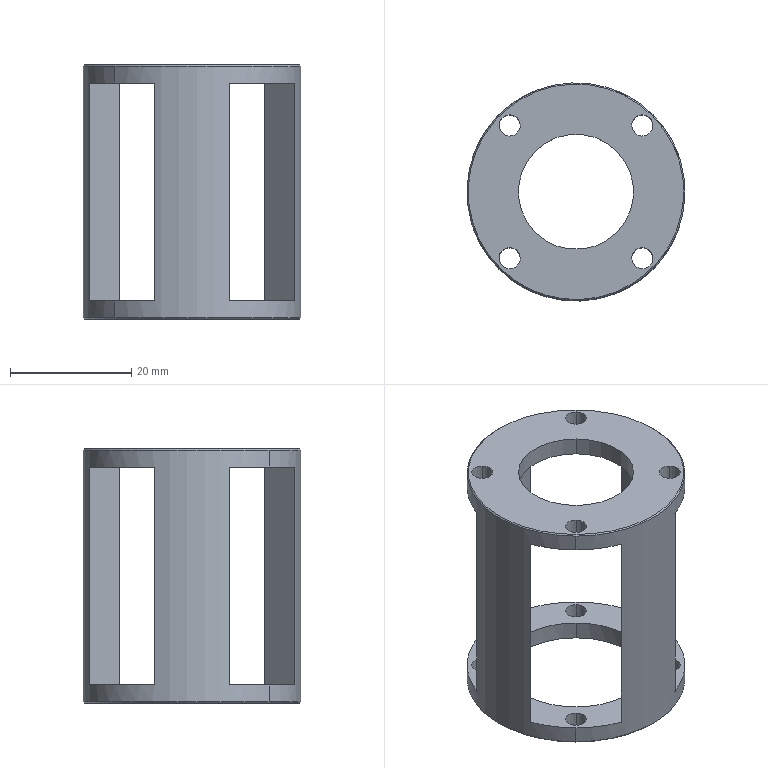Component | SolidWorks | MotorAssemblyWhen2-1_ConnectFastener2-1 | 1 solid | 41 faces | volume 10413 mm3 | cylinder 22 | plane 15 | cone 4 | commonest cylinder face diameters 3.5 x16 19.02 x2 36 x2 24 x2